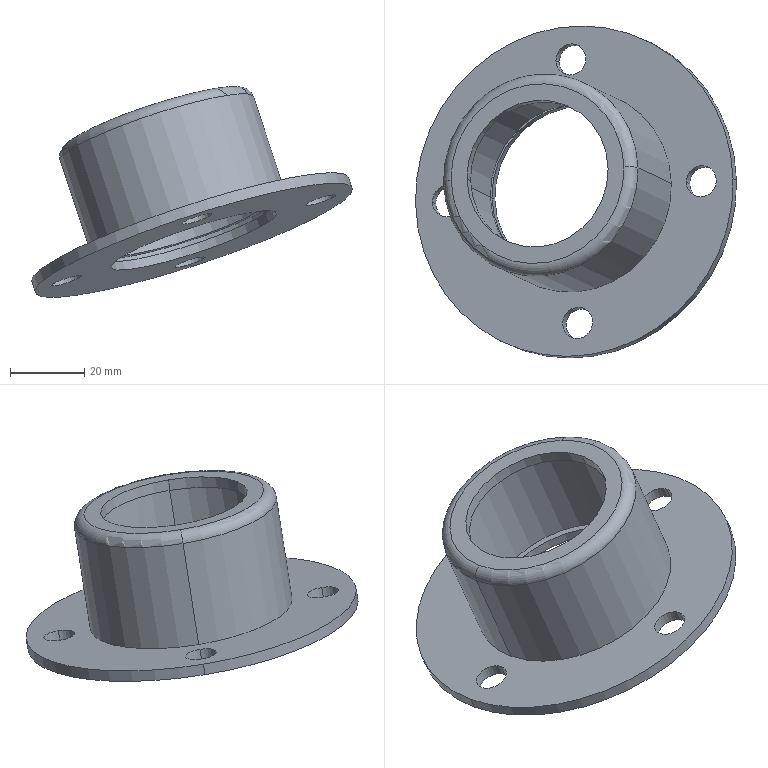Component | SolidWorks | FilmPressingSoilCoveringMechanism2Reverse-2_AttachedSoilDiskAssembly2-1_SoilDiskBearingHousing-1 | 1 solid | 28 faces | box 86.51 x 89.47 x 56.84 mm | volume 34355 mm3 | cylinder 20 | plane 6 | torus 2 | commonest cylinder face diameters 8.5 x8 47 x4 40 x2 55 x2 90 x2 51 x2
STEP:
#1=COLOUR_RGB('',0.7922,0.8196,0.9333);
#2=FILL_AREA_STYLE_COLOUR('',#1);
#3=FILL_AREA_STYLE('',(#2));
#4=SURFACE_STYLE_FILL_AREA(#3);
#5=SURFACE_SIDE_STYLE('',(#4));
#6=SURFACE_STYLE_USAGE(.BOTH.,#5);
#7=PRESENTATION_STYLE_ASSIGNMENT((#6));
#8=CARTESIAN_POINT('',(-74.256,-11.758,103.096));
#9=VERTEX_POINT('',#8);
#10=CARTESIAN_POINT('',(-74.574,-11.783,102.995));
#11=VERTEX_POINT('',#10);
#12=CARTESIAN_POINT('',(-74.415,-11.77,103.045));
#13=DIRECTION('',(-0.3093,0.1459,0.9397));
#14=DIRECTION('',(0.02532,-0.9865,0.1615));
#15=AXIS2_PLACEMENT_3D('',#12,#13,#14);
#16=CIRCLE('',#15,0.1673);
#17=EDGE_CURVE('',#9,#11,#16,.T.);
#18=ORIENTED_EDGE('',*,*,#17,.F.);
#19=CARTESIAN_POINT('',(-74.292,-11.741,103.207));
#20=VERTEX_POINT('',#19);
#21=CARTESIAN_POINT('',(-74.256,-11.758,103.096));
#22=DIRECTION('',(-0.3093,0.1459,0.9397));
#23=VECTOR('',#22,39.37);
#24=LINE('',#21,#23);
#25=EDGE_CURVE('',#9,#20,#24,.T.);
#26=ORIENTED_EDGE('',*,*,#25,.T.);
#27=CARTESIAN_POINT('',(-74.61,-11.765,103.106));
#28=VERTEX_POINT('',#27);
#29=CARTESIAN_POINT('',(-74.451,-11.753,103.156));
#30=DIRECTION('',(-0.3093,0.1459,0.9397));
#31=DIRECTION('',(0.02532,-0.9865,0.1615));
#32=AXIS2_PLACEMENT_3D('',#29,#30,#31);
#33=CIRCLE('',#32,0.1673);
#34=EDGE_CURVE('',#20,#28,#33,.T.);
#35=ORIENTED_EDGE('',*,*,#34,.T.);
#36=CARTESIAN_POINT('',(-74.574,-11.783,102.995));
#37=DIRECTION('',(-0.3093,0.1459,0.9397));
#38=VECTOR('',#37,39.37);
#39=LINE('',#36,#38);
#40=EDGE_CURVE('',#11,#28,#39,.T.);
#41=ORIENTED_EDGE('',*,*,#40,.F.);
#42=EDGE_LOOP('',(#18,#26,#35,#41));
#43=FACE_OUTER_BOUND('',#42,.T.);
#44=CARTESIAN_POINT('',(-74.415,-11.77,103.045));
#45=DIRECTION('',(-0.3093,0.1459,0.9397));
#46=DIRECTION('',(-0.9506,-0.07375,-0.3015));
#47=AXIS2_PLACEMENT_3D('',#44,#45,#46);
#48=CYLINDRICAL_SURFACE('',#47,0.1673);
#49=ADVANCED_FACE('',(#43),#48,.F.);
#50=CARTESIAN_POINT('',(-75.639,-10.464,102.44));
#51=VERTEX_POINT('',#50);
#52=CARTESIAN_POINT('',(-75.957,-10.489,102.339));
#53=VERTEX_POINT('',#52);
#54=CARTESIAN_POINT('',(-75.798,-10.477,102.389));
#55=DIRECTION('',(-0.3093,0.1459,0.9397));
#56=DIRECTION('',(0.9506,0.07375,0.3015));
#57=AXIS2_PLACEMENT_3D('',#54,#55,#56);
#58=CIRCLE('',#57,0.1673);
#59=EDGE_CURVE('',#51,#53,#58,.T.);
#60=ORIENTED_EDGE('',*,*,#59,.F.);
#61=CARTESIAN_POINT('',(-75.675,-10.447,102.551));
#62=VERTEX_POINT('',#61);
#63=CARTESIAN_POINT('',(-75.639,-10.464,102.44));
#64=DIRECTION('',(-0.3093,0.1459,0.9397));
#65=VECTOR('',#64,39.37);
#66=LINE('',#63,#65);
#67=EDGE_CURVE('',#51,#62,#66,.T.);
#68=ORIENTED_EDGE('',*,*,#67,.T.);
#69=CARTESIAN_POINT('',(-75.993,-10.472,102.45));
#70=VERTEX_POINT('',#69);
#71=CARTESIAN_POINT('',(-75.834,-10.459,102.5));
#72=DIRECTION('',(-0.3093,0.1459,0.9397));
#73=DIRECTION('',(0.9506,0.07375,0.3015));
#74=AXIS2_PLACEMENT_3D('',#71,#72,#73);
#75=CIRCLE('',#74,0.1673);
#76=EDGE_CURVE('',#62,#70,#75,.T.);
#77=ORIENTED_EDGE('',*,*,#76,.T.);
#78=CARTESIAN_POINT('',(-75.957,-10.489,102.339));
#79=DIRECTION('',(-0.3093,0.1459,0.9397));
#80=VECTOR('',#79,39.37);
#81=LINE('',#78,#80);
#82=EDGE_CURVE('',#53,#70,#81,.T.);
#83=ORIENTED_EDGE('',*,*,#82,.F.);
#84=EDGE_LOOP('',(#60,#68,#77,#83));
#85=FACE_OUTER_BOUND('',#84,.T.);
#86=CARTESIAN_POINT('',(-75.798,-10.477,102.389));
#87=DIRECTION('',(-0.3093,0.1459,0.9397));
#88=DIRECTION('',(-0.9506,-0.07375,-0.3015));
#89=AXIS2_PLACEMENT_3D('',#86,#87,#88);
#90=CYLINDRICAL_SURFACE('',#89,0.1673);
#91=ADVANCED_FACE('',(#85),#90,.F.);
#92=CARTESIAN_POINT('',(-76.95,-11.967,102.241));
#93=VERTEX_POINT('',#92);
#94=CARTESIAN_POINT('',(-77.268,-11.992,102.14));
#95=VERTEX_POINT('',#94);
#96=CARTESIAN_POINT('',(-77.109,-11.979,102.191));
#97=DIRECTION('',(-0.3093,0.1459,0.9397));
#98=DIRECTION('',(-0.02532,0.9865,-0.1615));
#99=AXIS2_PLACEMENT_3D('',#96,#97,#98);
#100=CIRCLE('',#99,0.1673);
#101=EDGE_CURVE('',#93,#95,#100,.T.);
#102=ORIENTED_EDGE('',*,*,#101,.F.);
#103=CARTESIAN_POINT('',(-76.987,-11.95,102.352));
#104=VERTEX_POINT('',#103);
#105=CARTESIAN_POINT('',(-76.95,-11.967,102.241));
#106=DIRECTION('',(-0.3093,0.1459,0.9397));
#107=VECTOR('',#106,39.37);
#108=LINE('',#105,#107);
#109=EDGE_CURVE('',#93,#104,#108,.T.);
#110=ORIENTED_EDGE('',*,*,#109,.T.);
#111=CARTESIAN_POINT('',(-77.305,-11.975,102.251));
#112=VERTEX_POINT('',#111);
#113=CARTESIAN_POINT('',(-77.146,-11.962,102.302));
#114=DIRECTION('',(-0.3093,0.1459,0.9397));
#115=DIRECTION('',(-0.02532,0.9865,-0.1615));
#116=AXIS2_PLACEMENT_3D('',#113,#114,#115);
#117=CIRCLE('',#116,0.1673);
#118=EDGE_CURVE('',#104,#112,#117,.T.);
#119=ORIENTED_EDGE('',*,*,#118,.T.);
#120=CARTESIAN_POINT('',(-77.268,-11.992,102.14));
#121=DIRECTION('',(-0.3093,0.1459,0.9397));
#122=VECTOR('',#121,39.37);
#123=LINE('',#120,#122);
#124=EDGE_CURVE('',#95,#112,#123,.T.);
#125=ORIENTED_EDGE('',*,*,#124,.F.);
#126=EDGE_LOOP('',(#102,#110,#119,#125));
#127=FACE_OUTER_BOUND('',#126,.T.);
#128=CARTESIAN_POINT('',(-77.109,-11.979,102.191));
#129=DIRECTION('',(-0.3093,0.1459,0.9397));
#130=DIRECTION('',(-0.9506,-0.07375,-0.3015));
#131=AXIS2_PLACEMENT_3D('',#128,#129,#130);
#132=CYLINDRICAL_SURFACE('',#131,0.1673);
#133=ADVANCED_FACE('',(#127),#132,.F.);
#134=CARTESIAN_POINT('',(-75.567,-13.261,102.897));
#135=VERTEX_POINT('',#134);
#136=CARTESIAN_POINT('',(-75.885,-13.285,102.797));
#137=VERTEX_POINT('',#136);
#138=CARTESIAN_POINT('',(-75.726,-13.273,102.847));
#139=DIRECTION('',(-0.3093,0.1459,0.9397));
#140=DIRECTION('',(-0.9506,-0.07375,-0.3015));
#141=AXIS2_PLACEMENT_3D('',#138,#139,#140);
#142=CIRCLE('',#141,0.1673);
#143=EDGE_CURVE('',#135,#137,#142,.T.);
#144=ORIENTED_EDGE('',*,*,#143,.F.);
#145=CARTESIAN_POINT('',(-75.604,-13.244,103.008));
#146=VERTEX_POINT('',#145);
#147=CARTESIAN_POINT('',(-75.567,-13.261,102.897));
#148=DIRECTION('',(-0.3093,0.1459,0.9397));
#149=VECTOR('',#148,39.37);
#150=LINE('',#147,#149);
#151=EDGE_CURVE('',#135,#146,#150,.T.);
#152=ORIENTED_EDGE('',*,*,#151,.T.);
#153=CARTESIAN_POINT('',(-75.922,-13.268,102.908));
#154=VERTEX_POINT('',#153);
#155=CARTESIAN_POINT('',(-75.763,-13.256,102.958));
#156=DIRECTION('',(-0.3093,0.1459,0.9397));
#157=DIRECTION('',(-0.9506,-0.07375,-0.3015));
#158=AXIS2_PLACEMENT_3D('',#155,#156,#157);
#159=CIRCLE('',#158,0.1673);
#160=EDGE_CURVE('',#146,#154,#159,.T.);
#161=ORIENTED_EDGE('',*,*,#160,.T.);
#162=CARTESIAN_POINT('',(-75.885,-13.285,102.797));
#163=DIRECTION('',(-0.3093,0.1459,0.9397));
#164=VECTOR('',#163,39.37);
#165=LINE('',#162,#164);
#166=EDGE_CURVE('',#137,#154,#165,.T.);
#167=ORIENTED_EDGE('',*,*,#166,.F.);
#168=EDGE_LOOP('',(#144,#152,#161,#167));
#169=FACE_OUTER_BOUND('',#168,.T.);
#170=CARTESIAN_POINT('',(-75.726,-13.273,102.847));
#171=DIRECTION('',(-0.3093,0.1459,0.9397));
#172=DIRECTION('',(-0.9506,-0.07375,-0.3015));
#173=AXIS2_PLACEMENT_3D('',#170,#171,#172);
#174=CYLINDRICAL_SURFACE('',#173,0.1673);
#175=ADVANCED_FACE('',(#169),#174,.F.);
#176=CARTESIAN_POINT('',(-76.937,-11.732,103.676));
#177=VERTEX_POINT('',#176);
#178=CARTESIAN_POINT('',(-75.44,-11.616,104.15));
#179=VERTEX_POINT('',#178);
#180=CARTESIAN_POINT('',(-76.188,-11.674,103.913));
#181=DIRECTION('',(0.3093,-0.1459,-0.9397));
#182=DIRECTION('',(0.9506,0.07375,0.3015));
#183=AXIS2_PLACEMENT_3D('',#180,#181,#182);
#184=CIRCLE('',#183,0.7874);
#185=EDGE_CURVE('',#177,#179,#184,.T.);
#186=ORIENTED_EDGE('',*,*,#185,.F.);
#187=CARTESIAN_POINT('',(-76.9,-11.749,103.565));
#188=VERTEX_POINT('',#187);
#189=CARTESIAN_POINT('',(-76.937,-11.732,103.676));
#190=DIRECTION('',(0.3093,-0.1459,-0.9397));
#191=VECTOR('',#190,39.37);
#192=LINE('',#189,#191);
#193=EDGE_CURVE('',#177,#188,#192,.T.);
#194=ORIENTED_EDGE('',*,*,#193,.T.);
#195=CARTESIAN_POINT('',(-75.403,-11.633,104.039));
#196=VERTEX_POINT('',#195);
#197=CARTESIAN_POINT('',(-76.152,-11.691,103.802));
#198=DIRECTION('',(0.3093,-0.1459,-0.9397));
#199=DIRECTION('',(0.9506,0.07375,0.3015));
#200=AXIS2_PLACEMENT_3D('',#197,#198,#199);
#201=CIRCLE('',#200,0.7874);
#202=EDGE_CURVE('',#188,#196,#201,.T.);
#203=ORIENTED_EDGE('',*,*,#202,.T.);
#204=CARTESIAN_POINT('',(-75.44,-11.616,104.15));
#205=DIRECTION('',(0.3093,-0.1459,-0.9397));
#206=VECTOR('',#205,39.37);
#207=LINE('',#204,#206);
#208=EDGE_CURVE('',#179,#196,#207,.T.);
#209=ORIENTED_EDGE('',*,*,#208,.F.);
#210=EDGE_LOOP('',(#186,#194,#203,#209));
#211=FACE_OUTER_BOUND('',#210,.T.);
#212=CARTESIAN_POINT('',(-76.188,-11.674,103.913));
#213=DIRECTION('',(0.3093,-0.1459,-0.9397));
#214=DIRECTION('',(0.9506,0.07375,0.3015));
#215=AXIS2_PLACEMENT_3D('',#212,#213,#214);
#216=CYLINDRICAL_SURFACE('',#215,0.7874);
#217=ADVANCED_FACE('',(#211),#216,.F.);
#218=CARTESIAN_POINT('',(-75.122,-11.611,104.128));
#219=VERTEX_POINT('',#218);
#220=CARTESIAN_POINT('',(-77.181,-11.771,103.476));
#221=VERTEX_POINT('',#220);
#222=CARTESIAN_POINT('',(-76.152,-11.691,103.802));
#223=DIRECTION('',(0.3093,-0.1459,-0.9397));
#224=DIRECTION('',(-0.9506,-0.07375,-0.3015));
#225=AXIS2_PLACEMENT_3D('',#222,#223,#224);
#226=CIRCLE('',#225,1.083);
#227=EDGE_CURVE('',#219,#221,#226,.T.);
#228=ORIENTED_EDGE('',*,*,#227,.F.);
#229=CARTESIAN_POINT('',(-75.271,-11.603,104.204));
#230=VERTEX_POINT('',#229);
#231=CARTESIAN_POINT('',(-75.235,-11.62,104.093));
#232=DIRECTION('',(0.02532,-0.9865,0.1615));
#233=DIRECTION('',(0.,-0.1616,-0.9869));
#234=AXIS2_PLACEMENT_3D('',#231,#232,#233);
#235=CIRCLE('',#234,0.1181);
#236=EDGE_CURVE('',#219,#230,#235,.T.);
#237=ORIENTED_EDGE('',*,*,#236,.T.);
#238=CARTESIAN_POINT('',(-77.105,-11.745,103.622));
#239=VERTEX_POINT('',#238);
#240=CARTESIAN_POINT('',(-76.188,-11.674,103.913));
#241=DIRECTION('',(-0.3093,0.1459,0.9397));
#242=DIRECTION('',(-0.9506,-0.07375,-0.3015));
#243=AXIS2_PLACEMENT_3D('',#240,#241,#242);
#244=CIRCLE('',#243,0.9646);
#245=EDGE_CURVE('',#239,#230,#244,.T.);
#246=ORIENTED_EDGE('',*,*,#245,.F.);
#247=CARTESIAN_POINT('',(-77.069,-11.762,103.511));
#248=DIRECTION('',(-0.02532,0.9865,-0.1615));
#249=DIRECTION('',(0.,0.1616,0.9869));
#250=AXIS2_PLACEMENT_3D('',#247,#248,#249);
#251=CIRCLE('',#250,0.1181);
#252=EDGE_CURVE('',#221,#239,#251,.T.);
#253=ORIENTED_EDGE('',*,*,#252,.F.);
#254=EDGE_LOOP('',(#228,#237,#246,#253));
#255=FACE_OUTER_BOUND('',#254,.T.);
#256=CARTESIAN_POINT('',(-76.152,-11.691,103.802));
#257=DIRECTION('',(-0.3093,0.1459,0.9397));
#258=DIRECTION('',(-0.9506,-0.07375,-0.3015));
#259=AXIS2_PLACEMENT_3D('',#256,#257,#258);
#260=TOROIDAL_SURFACE('',#259,0.9646,0.1181);
#261=ADVANCED_FACE('',(#255),#260,.T.);
#262=ORIENTED_EDGE('',*,*,#227,.T.);
#263=CARTESIAN_POINT('',(-76.828,-11.937,102.403));
#264=VERTEX_POINT('',#263);
#265=CARTESIAN_POINT('',(-77.217,-11.754,103.586));
#266=DIRECTION('',(0.3093,-0.1459,-0.9397));
#267=VECTOR('',#266,39.37);
#268=LINE('',#265,#267);
#269=EDGE_CURVE('',#221,#264,#268,.T.);
#270=ORIENTED_EDGE('',*,*,#269,.T.);
#271=CARTESIAN_POINT('',(-74.769,-11.778,103.055));
#272=VERTEX_POINT('',#271);
#273=CARTESIAN_POINT('',(-75.798,-11.858,102.729));
#274=DIRECTION('',(0.3093,-0.1459,-0.9397));
#275=DIRECTION('',(0.9506,0.07375,0.3015));
#276=AXIS2_PLACEMENT_3D('',#273,#274,#275);
#277=CIRCLE('',#276,1.083);
#278=EDGE_CURVE('',#272,#264,#277,.T.);
#279=ORIENTED_EDGE('',*,*,#278,.F.);
#280=CARTESIAN_POINT('',(-75.159,-11.594,104.239));
#281=DIRECTION('',(0.3093,-0.1459,-0.9397));
#282=VECTOR('',#281,39.37);
#283=LINE('',#280,#282);
#284=EDGE_CURVE('',#219,#272,#283,.T.);
#285=ORIENTED_EDGE('',*,*,#284,.F.);
#286=EDGE_LOOP('',(#262,#270,#279,#285));
#287=FACE_OUTER_BOUND('',#286,.T.);
#288=CARTESIAN_POINT('',(-76.188,-11.674,103.913));
#289=DIRECTION('',(0.3093,-0.1459,-0.9397));
#290=DIRECTION('',(0.9506,0.07375,0.3015));
#291=AXIS2_PLACEMENT_3D('',#288,#289,#290);
#292=CYLINDRICAL_SURFACE('',#291,1.083);
#293=ADVANCED_FACE('',(#287),#292,.T.);
#294=CARTESIAN_POINT('',(-74.114,-11.727,103.263));
#295=VERTEX_POINT('',#294);
#296=CARTESIAN_POINT('',(-77.483,-11.988,102.195));
#297=VERTEX_POINT('',#296);
#298=CARTESIAN_POINT('',(-75.798,-11.858,102.729));
#299=DIRECTION('',(0.3093,-0.1459,-0.9397));
#300=DIRECTION('',(0.9506,0.07375,0.3015));
#301=AXIS2_PLACEMENT_3D('',#298,#299,#300);
#302=CIRCLE('',#301,1.772);
#303=EDGE_CURVE('',#295,#297,#302,.T.);
#304=ORIENTED_EDGE('',*,*,#303,.T.);
#305=CARTESIAN_POINT('',(-77.446,-12.006,102.084));
#306=VERTEX_POINT('',#305);
#307=CARTESIAN_POINT('',(-77.483,-11.988,102.195));
#308=DIRECTION('',(0.3093,-0.1459,-0.9397));
#309=VECTOR('',#308,39.37);
#310=LINE('',#307,#309);
#311=EDGE_CURVE('',#297,#306,#310,.T.);
#312=ORIENTED_EDGE('',*,*,#311,.T.);
#313=CARTESIAN_POINT('',(-74.078,-11.744,103.152));
#314=VERTEX_POINT('',#313);
#315=CARTESIAN_POINT('',(-75.762,-11.875,102.618));
#316=DIRECTION('',(0.3093,-0.1459,-0.9397));
#317=DIRECTION('',(0.9506,0.07375,0.3015));
#318=AXIS2_PLACEMENT_3D('',#315,#316,#317);
#319=CIRCLE('',#318,1.772);
#320=EDGE_CURVE('',#314,#306,#319,.T.);
#321=ORIENTED_EDGE('',*,*,#320,.F.);
#322=CARTESIAN_POINT('',(-74.114,-11.727,103.263));
#323=DIRECTION('',(0.3093,-0.1459,-0.9397));
#324=VECTOR('',#323,39.37);
#325=LINE('',#322,#324);
#326=EDGE_CURVE('',#295,#314,#325,.T.);
#327=ORIENTED_EDGE('',*,*,#326,.F.);
#328=EDGE_LOOP('',(#304,#312,#321,#327));
#329=FACE_OUTER_BOUND('',#328,.T.);
#330=CARTESIAN_POINT('',(-75.798,-11.858,102.729));
#331=DIRECTION('',(0.3093,-0.1459,-0.9397));
#332=DIRECTION('',(0.9506,0.07375,0.3015));
#333=AXIS2_PLACEMENT_3D('',#330,#331,#332);
#334=CYLINDRICAL_SURFACE('',#333,1.772);
#335=ADVANCED_FACE('',(#329),#334,.T.);
#336=CARTESIAN_POINT('',(-77.031,-11.759,103.523));
#337=VERTEX_POINT('',#336);
#338=CARTESIAN_POINT('',(-75.272,-11.623,104.081));
#339=VERTEX_POINT('',#338);
#340=CARTESIAN_POINT('',(-76.152,-11.691,103.802));
#341=DIRECTION('',(0.3093,-0.1459,-0.9397));
#342=DIRECTION('',(0.9506,0.07375,0.3015));
#343=AXIS2_PLACEMENT_3D('',#340,#341,#342);
#344=CIRCLE('',#343,0.9252);
#345=EDGE_CURVE('',#337,#339,#344,.T.);
#346=ORIENTED_EDGE('',*,*,#345,.F.);
#347=CARTESIAN_POINT('',(-76.69,-11.92,102.487));
#348=VERTEX_POINT('',#347);
#349=CARTESIAN_POINT('',(-77.031,-11.759,103.523));
#350=DIRECTION('',(0.3093,-0.1459,-0.9397));
#351=VECTOR('',#350,39.37);
#352=LINE('',#349,#351);
#353=EDGE_CURVE('',#337,#348,#352,.T.);
#354=ORIENTED_EDGE('',*,*,#353,.T.);
#355=CARTESIAN_POINT('',(-74.931,-11.784,103.045));
#356=VERTEX_POINT('',#355);
#357=CARTESIAN_POINT('',(-75.811,-11.852,102.766));
#358=DIRECTION('',(0.3093,-0.1459,-0.9397));
#359=DIRECTION('',(-0.9506,-0.07375,-0.3015));
#360=AXIS2_PLACEMENT_3D('',#357,#358,#359);
#361=CIRCLE('',#360,0.9252);
#362=EDGE_CURVE('',#348,#356,#361,.T.);
#363=ORIENTED_EDGE('',*,*,#362,.T.);
#364=CARTESIAN_POINT('',(-75.272,-11.623,104.081));
#365=DIRECTION('',(0.3093,-0.1459,-0.9397));
#366=VECTOR('',#365,39.37);
#367=LINE('',#364,#366);
#368=EDGE_CURVE('',#339,#356,#367,.T.);
#369=ORIENTED_EDGE('',*,*,#368,.F.);
#370=EDGE_LOOP('',(#346,#354,#363,#369));
#371=FACE_OUTER_BOUND('',#370,.T.);
#372=CARTESIAN_POINT('',(-76.152,-11.691,103.802));
#373=DIRECTION('',(0.3093,-0.1459,-0.9397));
#374=DIRECTION('',(0.9506,0.07375,0.3015));
#375=AXIS2_PLACEMENT_3D('',#372,#373,#374);
#376=CYLINDRICAL_SURFACE('',#375,0.9252);
#377=ADVANCED_FACE('',(#371),#376,.F.);
#378=CARTESIAN_POINT('',(-76.765,-11.926,102.463));
#379=VERTEX_POINT('',#378);
#380=CARTESIAN_POINT('',(-74.856,-11.778,103.069));
#381=VERTEX_POINT('',#380);
#382=CARTESIAN_POINT('',(-75.811,-11.852,102.766));
#383=DIRECTION('',(0.3093,-0.1459,-0.9397));
#384=DIRECTION('',(0.9506,0.07375,0.3015));
#385=AXIS2_PLACEMENT_3D('',#382,#383,#384);
#386=CIRCLE('',#385,1.004);
#387=EDGE_CURVE('',#379,#381,#386,.T.);
#388=ORIENTED_EDGE('',*,*,#387,.F.);
#389=CARTESIAN_POINT('',(-76.747,-11.935,102.408));
#390=VERTEX_POINT('',#389);
#391=CARTESIAN_POINT('',(-76.716,-11.949,102.315));
#392=DIRECTION('',(0.3093,-0.1459,-0.9397));
#393=VECTOR('',#392,39.37);
#394=LINE('',#391,#393);
#395=EDGE_CURVE('',#379,#390,#394,.T.);
#396=ORIENTED_EDGE('',*,*,#395,.T.);
#397=CARTESIAN_POINT('',(-74.838,-11.786,103.013));
#398=VERTEX_POINT('',#397);
#399=CARTESIAN_POINT('',(-75.792,-11.861,102.711));
#400=DIRECTION('',(0.3093,-0.1459,-0.9397));
#401=DIRECTION('',(0.9506,0.07375,0.3015));
#402=AXIS2_PLACEMENT_3D('',#399,#400,#401);
#403=CIRCLE('',#402,1.004);
#404=EDGE_CURVE('',#390,#398,#403,.T.);
#405=ORIENTED_EDGE('',*,*,#404,.T.);
#406=CARTESIAN_POINT('',(-74.808,-11.801,102.921));
#407=DIRECTION('',(0.3093,-0.1459,-0.9397));
#408=VECTOR('',#407,39.37);
#409=LINE('',#406,#408);
#410=EDGE_CURVE('',#381,#398,#409,.T.);
#411=ORIENTED_EDGE('',*,*,#410,.F.);
#412=EDGE_LOOP('',(#388,#396,#405,#411));
#413=FACE_OUTER_BOUND('',#412,.T.);
#414=CARTESIAN_POINT('',(-75.762,-11.875,102.618));
#415=DIRECTION('',(0.3093,-0.1459,-0.9397));
#416=DIRECTION('',(0.9506,0.07375,0.3015));
#417=AXIS2_PLACEMENT_3D('',#414,#415,#416);
#418=CYLINDRICAL_SURFACE('',#417,1.004);
#419=ADVANCED_FACE('',(#413),#418,.F.);
#420=CARTESIAN_POINT('',(-74.913,-11.792,102.989));
#421=VERTEX_POINT('',#420);
#422=CARTESIAN_POINT('',(-76.672,-11.929,102.432));
#423=VERTEX_POINT('',#422);
#424=CARTESIAN_POINT('',(-75.792,-11.861,102.711));
#425=DIRECTION('',(-0.3093,0.1459,0.9397));
#426=DIRECTION('',(0.9506,0.07375,0.3015));
#427=AXIS2_PLACEMENT_3D('',#424,#425,#426);
#428=CIRCLE('',#427,0.9252);
#429=EDGE_CURVE('',#421,#423,#428,.T.);
#430=ORIENTED_EDGE('',*,*,#429,.T.);
#431=CARTESIAN_POINT('',(-76.641,-11.943,102.339));
#432=VERTEX_POINT('',#431);
#433=CARTESIAN_POINT('',(-77.031,-11.759,103.523));
#434=DIRECTION('',(0.3093,-0.1459,-0.9397));
#435=VECTOR('',#434,39.37);
#436=LINE('',#433,#435);
#437=EDGE_CURVE('',#423,#432,#436,.T.);
#438=ORIENTED_EDGE('',*,*,#437,.T.);
#439=CARTESIAN_POINT('',(-74.882,-11.807,102.897));
#440=VERTEX_POINT('',#439);
#441=CARTESIAN_POINT('',(-75.762,-11.875,102.618));
#442=DIRECTION('',(0.3093,-0.1459,-0.9397));
#443=DIRECTION('',(0.9506,0.07375,0.3015));
#444=AXIS2_PLACEMENT_3D('',#441,#442,#443);
#445=CIRCLE('',#444,0.9252);
#446=EDGE_CURVE('',#432,#440,#445,.T.);
#447=ORIENTED_EDGE('',*,*,#446,.T.);
#448=CARTESIAN_POINT('',(-75.272,-11.623,104.081));
#449=DIRECTION('',(0.3093,-0.1459,-0.9397));
#450=VECTOR('',#449,39.37);
#451=LINE('',#448,#450);
#452=EDGE_CURVE('',#421,#440,#451,.T.);
#453=ORIENTED_EDGE('',*,*,#452,.F.);
#454=EDGE_LOOP('',(#430,#438,#447,#453));
#455=FACE_OUTER_BOUND('',#454,.T.);
#456=CARTESIAN_POINT('',(-76.152,-11.691,103.802));
#457=DIRECTION('',(0.3093,-0.1459,-0.9397));
#458=DIRECTION('',(0.9506,0.07375,0.3015));
#459=AXIS2_PLACEMENT_3D('',#456,#457,#458);
#460=CYLINDRICAL_SURFACE('',#459,0.9252);
#461=ADVANCED_FACE('',(#455),#460,.F.);
#462=CARTESIAN_POINT('',(-74.415,-11.77,103.045));
#463=DIRECTION('',(-0.3093,0.1459,0.9397));
#464=DIRECTION('',(0.02532,-0.9865,0.1615));
#465=AXIS2_PLACEMENT_3D('',#462,#463,#464);
#466=CIRCLE('',#465,0.1673);
#467=EDGE_CURVE('',#11,#9,#466,.T.);
#468=ORIENTED_EDGE('',*,*,#467,.T.);
#469=ORIENTED_EDGE('',*,*,#17,.T.);
#470=EDGE_LOOP('',(#468,#469));
#471=FACE_BOUND('',#470,.T.);
#472=CARTESIAN_POINT('',(-75.798,-10.477,102.389));
#473=DIRECTION('',(-0.3093,0.1459,0.9397));
#474=DIRECTION('',(0.9506,0.07375,0.3015));
#475=AXIS2_PLACEMENT_3D('',#472,#473,#474);
#476=CIRCLE('',#475,0.1673);
#477=EDGE_CURVE('',#53,#51,#476,.T.);
#478=ORIENTED_EDGE('',*,*,#477,.T.);
#479=ORIENTED_EDGE('',*,*,#59,.T.);
#480=EDGE_LOOP('',(#478,#479));
#481=FACE_BOUND('',#480,.T.);
#482=CARTESIAN_POINT('',(-77.109,-11.979,102.191));
#483=DIRECTION('',(-0.3093,0.1459,0.9397));
#484=DIRECTION('',(-0.02532,0.9865,-0.1615));
#485=AXIS2_PLACEMENT_3D('',#482,#483,#484);
#486=CIRCLE('',#485,0.1673);
#487=EDGE_CURVE('',#95,#93,#486,.T.);
#488=ORIENTED_EDGE('',*,*,#487,.T.);
#489=ORIENTED_EDGE('',*,*,#101,.T.);
#490=EDGE_LOOP('',(#488,#489));
#491=FACE_BOUND('',#490,.T.);
#492=CARTESIAN_POINT('',(-75.726,-13.273,102.847));
#493=DIRECTION('',(-0.3093,0.1459,0.9397));
#494=DIRECTION('',(-0.9506,-0.07375,-0.3015));
#495=AXIS2_PLACEMENT_3D('',#492,#493,#494);
#496=CIRCLE('',#495,0.1673);
#497=EDGE_CURVE('',#137,#135,#496,.T.);
#498=ORIENTED_EDGE('',*,*,#497,.T.);
#499=ORIENTED_EDGE('',*,*,#143,.T.);
#500=EDGE_LOOP('',(#498,#499));
#501=FACE_BOUND('',#500,.T.);
#502=CARTESIAN_POINT('',(-75.762,-11.875,102.618));
#503=DIRECTION('',(0.3093,-0.1459,-0.9397));
#504=DIRECTION('',(0.9506,0.07375,0.3015));
#505=AXIS2_PLACEMENT_3D('',#502,#503,#504);
#506=CIRCLE('',#505,0.9252);
#507=EDGE_CURVE('',#440,#432,#506,.T.);
#508=ORIENTED_EDGE('',*,*,#507,.F.);
#509=ORIENTED_EDGE('',*,*,#446,.F.);
#510=EDGE_LOOP('',(#508,#509));
#511=FACE_BOUND('',#510,.T.);
#512=ORIENTED_EDGE('',*,*,#320,.T.);
#513=CARTESIAN_POINT('',(-75.762,-11.875,102.618));
#514=DIRECTION('',(0.3093,-0.1459,-0.9397));
#515=DIRECTION('',(0.9506,0.07375,0.3015));
#516=AXIS2_PLACEMENT_3D('',#513,#514,#515);
#517=CIRCLE('',#516,1.772);
#518=EDGE_CURVE('',#306,#314,#517,.T.);
#519=ORIENTED_EDGE('',*,*,#518,.T.);
#520=EDGE_LOOP('',(#512,#519));
#521=FACE_OUTER_BOUND('',#520,.T.);
#522=CARTESIAN_POINT('',(-75.762,-11.875,102.618));
#523=DIRECTION('',(-0.3093,0.1459,0.9397));
#524=DIRECTION('',(-0.9506,-0.07375,-0.3015));
#525=AXIS2_PLACEMENT_3D('',#522,#523,#524);
#526=PLANE('',#525);
#527=ADVANCED_FACE('',(#471,#481,#491,#501,#511,#521),#526,.F.);
#528=ORIENTED_EDGE('',*,*,#437,.F.);
#529=CARTESIAN_POINT('',(-75.792,-11.861,102.711));
#530=DIRECTION('',(-0.3093,0.1459,0.9397));
#531=DIRECTION('',(0.9506,0.07375,0.3015));
#532=AXIS2_PLACEMENT_3D('',#529,#530,#531);
#533=CIRCLE('',#532,0.9252);
#534=EDGE_CURVE('',#423,#421,#533,.T.);
#535=ORIENTED_EDGE('',*,*,#534,.T.);
#536=ORIENTED_EDGE('',*,*,#452,.T.);
#537=ORIENTED_EDGE('',*,*,#507,.T.);
#538=EDGE_LOOP('',(#528,#535,#536,#537));
#539=FACE_OUTER_BOUND('',#538,.T.);
#540=CARTESIAN_POINT('',(-76.152,-11.691,103.802));
#541=DIRECTION('',(0.3093,-0.1459,-0.9397));
#542=DIRECTION('',(0.9506,0.07375,0.3015));
#543=AXIS2_PLACEMENT_3D('',#540,#541,#542);
#544=CYLINDRICAL_SURFACE('',#543,0.9252);
#545=ADVANCED_FACE('',(#539),#544,.F.);
#546=CARTESIAN_POINT('',(-75.811,-11.852,102.766));
#547=DIRECTION('',(0.3093,-0.1459,-0.9397));
#548=DIRECTION('',(0.9506,0.07375,0.3015));
#549=AXIS2_PLACEMENT_3D('',#546,#547,#548);
#550=CIRCLE('',#549,1.004);
#551=EDGE_CURVE('',#381,#379,#550,.T.);
#552=ORIENTED_EDGE('',*,*,#551,.T.);
#553=ORIENTED_EDGE('',*,*,#387,.T.);
#554=EDGE_LOOP('',(#552,#553));
#555=FACE_OUTER_BOUND('',#554,.T.);
#556=CARTESIAN_POINT('',(-75.811,-11.852,102.766));
#557=DIRECTION('',(0.3093,-0.1459,-0.9397));
#558=DIRECTION('',(-0.9506,-0.07375,-0.3015));
#559=AXIS2_PLACEMENT_3D('',#556,#557,#558);
#560=CIRCLE('',#559,0.9252);
#561=EDGE_CURVE('',#356,#348,#560,.T.);
#562=ORIENTED_EDGE('',*,*,#561,.F.);
#563=ORIENTED_EDGE('',*,*,#362,.F.);
#564=EDGE_LOOP('',(#562,#563));
#565=FACE_BOUND('',#564,.T.);
#566=CARTESIAN_POINT('',(-74.856,-11.778,103.069));
#567=DIRECTION('',(-0.3093,0.1459,0.9397));
#568=DIRECTION('',(-0.9506,-0.07375,-0.3015));
#569=AXIS2_PLACEMENT_3D('',#566,#567,#568);
#570=PLANE('',#569);
#571=ADVANCED_FACE('',(#555,#565),#570,.F.);
#572=CARTESIAN_POINT('',(-75.792,-11.861,102.711));
#573=DIRECTION('',(0.3093,-0.1459,-0.9397));
#574=DIRECTION('',(0.9506,0.07375,0.3015));
#575=AXIS2_PLACEMENT_3D('',#572,#573,#574);
#576=CIRCLE('',#575,1.004);
#577=EDGE_CURVE('',#398,#390,#576,.T.);
#578=ORIENTED_EDGE('',*,*,#577,.F.);
#579=ORIENTED_EDGE('',*,*,#404,.F.);
#580=EDGE_LOOP('',(#578,#579));
#581=FACE_OUTER_BOUND('',#580,.T.);
#582=ORIENTED_EDGE('',*,*,#429,.F.);
#583=ORIENTED_EDGE('',*,*,#534,.F.);
#584=EDGE_LOOP('',(#582,#583));
#585=FACE_BOUND('',#584,.T.);
#586=CARTESIAN_POINT('',(-74.838,-11.786,103.013));
#587=DIRECTION('',(0.3093,-0.1459,-0.9397));
#588=DIRECTION('',(0.9506,0.07375,0.3015));
#589=AXIS2_PLACEMENT_3D('',#586,#587,#588);
#590=PLANE('',#589);
#591=ADVANCED_FACE('',(#581,#585),#590,.F.);
#592=ORIENTED_EDGE('',*,*,#395,.F.);
#593=ORIENTED_EDGE('',*,*,#551,.F.);
#594=ORIENTED_EDGE('',*,*,#410,.T.);
#595=ORIENTED_EDGE('',*,*,#577,.T.);
#596=EDGE_LOOP('',(#592,#593,#594,#595));
#597=FACE_OUTER_BOUND('',#596,.T.);
#598=CARTESIAN_POINT('',(-75.762,-11.875,102.618));
#599=DIRECTION('',(0.3093,-0.1459,-0.9397));
#600=DIRECTION('',(0.9506,0.07375,0.3015));
#601=AXIS2_PLACEMENT_3D('',#598,#599,#600);
#602=CYLINDRICAL_SURFACE('',#601,1.004);
#603=ADVANCED_FACE('',(#597),#602,.F.);
#604=CARTESIAN_POINT('',(-76.152,-11.691,103.802));
#605=DIRECTION('',(0.3093,-0.1459,-0.9397));
#606=DIRECTION('',(0.9506,0.07375,0.3015));
#607=AXIS2_PLACEMENT_3D('',#604,#605,#606);
#608=CIRCLE('',#607,0.7874);
#609=EDGE_CURVE('',#196,#188,#608,.T.);
#610=ORIENTED_EDGE('',*,*,#609,.F.);
#611=ORIENTED_EDGE('',*,*,#202,.F.);
#612=EDGE_LOOP('',(#610,#611));
#613=FACE_BOUND('',#612,.T.);
#614=CARTESIAN_POINT('',(-76.152,-11.691,103.802));
#615=DIRECTION('',(0.3093,-0.1459,-0.9397));
#616=DIRECTION('',(0.9506,0.07375,0.3015));
#617=AXIS2_PLACEMENT_3D('',#614,#615,#616);
#618=CIRCLE('',#617,0.9252);
#619=EDGE_CURVE('',#339,#337,#618,.T.);
#620=ORIENTED_EDGE('',*,*,#619,.T.);
#621=ORIENTED_EDGE('',*,*,#345,.T.);
#622=EDGE_LOOP('',(#620,#621));
#623=FACE_OUTER_BOUND('',#622,.T.);
#624=CARTESIAN_POINT('',(-76.152,-11.691,103.802));
#625=DIRECTION('',(0.3093,-0.1459,-0.9397));
#626=DIRECTION('',(0.9506,0.07375,0.3015));
#627=AXIS2_PLACEMENT_3D('',#624,#625,#626);
#628=PLANE('',#627);
#629=ADVANCED_FACE('',(#613,#623),#628,.T.);
#630=ORIENTED_EDGE('',*,*,#353,.F.);
#631=ORIENTED_EDGE('',*,*,#619,.F.);
#632=ORIENTED_EDGE('',*,*,#368,.T.);
#633=ORIENTED_EDGE('',*,*,#561,.T.);
#634=EDGE_LOOP('',(#630,#631,#632,#633));
#635=FACE_OUTER_BOUND('',#634,.T.);
#636=CARTESIAN_POINT('',(-76.152,-11.691,103.802));
#637=DIRECTION('',(0.3093,-0.1459,-0.9397));
#638=DIRECTION('',(0.9506,0.07375,0.3015));
#639=AXIS2_PLACEMENT_3D('',#636,#637,#638);
#640=CYLINDRICAL_SURFACE('',#639,0.9252);
#641=ADVANCED_FACE('',(#635),#640,.F.);
#642=ORIENTED_EDGE('',*,*,#311,.F.);
#643=CARTESIAN_POINT('',(-75.798,-11.858,102.729));
#644=DIRECTION('',(0.3093,-0.1459,-0.9397));
#645=DIRECTION('',(0.9506,0.07375,0.3015));
#646=AXIS2_PLACEMENT_3D('',#643,#644,#645);
#647=CIRCLE('',#646,1.772);
#648=EDGE_CURVE('',#297,#295,#647,.T.);
#649=ORIENTED_EDGE('',*,*,#648,.T.);
#650=ORIENTED_EDGE('',*,*,#326,.T.);
#651=ORIENTED_EDGE('',*,*,#518,.F.);
#652=EDGE_LOOP('',(#642,#649,#650,#651));
#653=FACE_OUTER_BOUND('',#652,.T.);
#654=CARTESIAN_POINT('',(-75.798,-11.858,102.729));
#655=DIRECTION('',(0.3093,-0.1459,-0.9397));
#656=DIRECTION('',(0.9506,0.07375,0.3015));
#657=AXIS2_PLACEMENT_3D('',#654,#655,#656);
#658=CYLINDRICAL_SURFACE('',#657,1.772);
#659=ADVANCED_FACE('',(#653),#658,.T.);
#660=CARTESIAN_POINT('',(-74.451,-11.753,103.156));
#661=DIRECTION('',(-0.3093,0.1459,0.9397));
#662=DIRECTION('',(0.02532,-0.9865,0.1615));
#663=AXIS2_PLACEMENT_3D('',#660,#661,#662);
#664=CIRCLE('',#663,0.1673);
#665=EDGE_CURVE('',#28,#20,#664,.T.);
#666=ORIENTED_EDGE('',*,*,#665,.F.);
#667=ORIENTED_EDGE('',*,*,#34,.F.);
#668=EDGE_LOOP('',(#666,#667));
#669=FACE_BOUND('',#668,.T.);
#670=CARTESIAN_POINT('',(-75.834,-10.459,102.5));
#671=DIRECTION('',(-0.3093,0.1459,0.9397));
#672=DIRECTION('',(0.9506,0.07375,0.3015));
#673=AXIS2_PLACEMENT_3D('',#670,#671,#672);
#674=CIRCLE('',#673,0.1673);
#675=EDGE_CURVE('',#70,#62,#674,.T.);
#676=ORIENTED_EDGE('',*,*,#675,.F.);
#677=ORIENTED_EDGE('',*,*,#76,.F.);
#678=EDGE_LOOP('',(#676,#677));
#679=FACE_BOUND('',#678,.T.);
#680=CARTESIAN_POINT('',(-77.146,-11.962,102.302));
#681=DIRECTION('',(-0.3093,0.1459,0.9397));
#682=DIRECTION('',(-0.02532,0.9865,-0.1615));
#683=AXIS2_PLACEMENT_3D('',#680,#681,#682);
#684=CIRCLE('',#683,0.1673);
#685=EDGE_CURVE('',#112,#104,#684,.T.);
#686=ORIENTED_EDGE('',*,*,#685,.F.);
#687=ORIENTED_EDGE('',*,*,#118,.F.);
#688=EDGE_LOOP('',(#686,#687));
#689=FACE_BOUND('',#688,.T.);
#690=CARTESIAN_POINT('',(-75.763,-13.256,102.958));
#691=DIRECTION('',(-0.3093,0.1459,0.9397));
#692=DIRECTION('',(-0.9506,-0.07375,-0.3015));
#693=AXIS2_PLACEMENT_3D('',#690,#691,#692);
#694=CIRCLE('',#693,0.1673);
#695=EDGE_CURVE('',#154,#146,#694,.T.);
#696=ORIENTED_EDGE('',*,*,#695,.F.);
#697=ORIENTED_EDGE('',*,*,#160,.F.);
#698=EDGE_LOOP('',(#696,#697));
#699=FACE_BOUND('',#698,.T.);
#700=ORIENTED_EDGE('',*,*,#278,.T.);
#701=CARTESIAN_POINT('',(-75.798,-11.858,102.729));
#702=DIRECTION('',(0.3093,-0.1459,-0.9397));
#703=DIRECTION('',(0.9506,0.07375,0.3015));
#704=AXIS2_PLACEMENT_3D('',#701,#702,#703);
#705=CIRCLE('',#704,1.083);
#706=EDGE_CURVE('',#264,#272,#705,.T.);
#707=ORIENTED_EDGE('',*,*,#706,.T.);
#708=EDGE_LOOP('',(#700,#707));
#709=FACE_BOUND('',#708,.T.);
#710=ORIENTED_EDGE('',*,*,#303,.F.);
#711=ORIENTED_EDGE('',*,*,#648,.F.);
#712=EDGE_LOOP('',(#710,#711));
#713=FACE_OUTER_BOUND('',#712,.T.);
#714=CARTESIAN_POINT('',(-75.798,-11.858,102.729));
#715=DIRECTION('',(0.3093,-0.1459,-0.9397));
#716=DIRECTION('',(0.9506,0.07375,0.3015));
#717=AXIS2_PLACEMENT_3D('',#714,#715,#716);
#718=PLANE('',#717);
#719=ADVANCED_FACE('',(#669,#679,#689,#699,#709,#713),#718,.F.);
#720=CARTESIAN_POINT('',(-76.188,-11.674,103.913));
#721=DIRECTION('',(0.3093,-0.1459,-0.9397));
#722=DIRECTION('',(0.9506,0.07375,0.3015));
#723=AXIS2_PLACEMENT_3D('',#720,#721,#722);
#724=CIRCLE('',#723,0.7874);
#725=EDGE_CURVE('',#179,#177,#724,.T.);
#726=ORIENTED_EDGE('',*,*,#725,.T.);
#727=ORIENTED_EDGE('',*,*,#185,.T.);
#728=EDGE_LOOP('',(#726,#727));
#729=FACE_BOUND('',#728,.T.);
#730=ORIENTED_EDGE('',*,*,#245,.T.);
#731=CARTESIAN_POINT('',(-76.188,-11.674,103.913));
#732=DIRECTION('',(-0.3093,0.1459,0.9397));
#733=DIRECTION('',(-0.9506,-0.07375,-0.3015));
#734=AXIS2_PLACEMENT_3D('',#731,#732,#733);
#735=CIRCLE('',#734,0.9646);
#736=EDGE_CURVE('',#230,#239,#735,.T.);
#737=ORIENTED_EDGE('',*,*,#736,.T.);
#738=EDGE_LOOP('',(#730,#737));
#739=FACE_OUTER_BOUND('',#738,.T.);
#740=CARTESIAN_POINT('',(-76.188,-11.674,103.913));
#741=DIRECTION('',(-0.3093,0.1459,0.9397));
#742=DIRECTION('',(-0.9506,-0.07375,-0.3015));
#743=AXIS2_PLACEMENT_3D('',#740,#741,#742);
#744=PLANE('',#743);
#745=ADVANCED_FACE('',(#729,#739),#744,.T.);
#746=ORIENTED_EDGE('',*,*,#269,.F.);
#747=CARTESIAN_POINT('',(-76.152,-11.691,103.802));
#748=DIRECTION('',(0.3093,-0.1459,-0.9397));
#749=DIRECTION('',(-0.9506,-0.07375,-0.3015));
#750=AXIS2_PLACEMENT_3D('',#747,#748,#749);
#751=CIRCLE('',#750,1.083);
#752=EDGE_CURVE('',#221,#219,#751,.T.);
#753=ORIENTED_EDGE('',*,*,#752,.T.);
#754=ORIENTED_EDGE('',*,*,#284,.T.);
#755=ORIENTED_EDGE('',*,*,#706,.F.);
#756=EDGE_LOOP('',(#746,#753,#754,#755));
#757=FACE_OUTER_BOUND('',#756,.T.);
#758=CARTESIAN_POINT('',(-76.188,-11.674,103.913));
#759=DIRECTION('',(0.3093,-0.1459,-0.9397));
#760=DIRECTION('',(0.9506,0.07375,0.3015));
#761=AXIS2_PLACEMENT_3D('',#758,#759,#760);
#762=CYLINDRICAL_SURFACE('',#761,1.083);
#763=ADVANCED_FACE('',(#757),#762,.T.);
#764=ORIENTED_EDGE('',*,*,#236,.F.);
#765=ORIENTED_EDGE('',*,*,#752,.F.);
#766=ORIENTED_EDGE('',*,*,#252,.T.);
#767=ORIENTED_EDGE('',*,*,#736,.F.);
#768=EDGE_LOOP('',(#764,#765,#766,#767));
#769=FACE_OUTER_BOUND('',#768,.T.);
#770=CARTESIAN_POINT('',(-76.152,-11.691,103.802));
#771=DIRECTION('',(-0.3093,0.1459,0.9397));
#772=DIRECTION('',(-0.9506,-0.07375,-0.3015));
#773=AXIS2_PLACEMENT_3D('',#770,#771,#772);
#774=TOROIDAL_SURFACE('',#773,0.9646,0.1181);
#775=ADVANCED_FACE('',(#769),#774,.T.);
#776=ORIENTED_EDGE('',*,*,#193,.F.);
#777=ORIENTED_EDGE('',*,*,#725,.F.);
#778=ORIENTED_EDGE('',*,*,#208,.T.);
#779=ORIENTED_EDGE('',*,*,#609,.T.);
#780=EDGE_LOOP('',(#776,#777,#778,#779));
#781=FACE_OUTER_BOUND('',#780,.T.);
#782=CARTESIAN_POINT('',(-76.188,-11.674,103.913));
#783=DIRECTION('',(0.3093,-0.1459,-0.9397));
#784=DIRECTION('',(0.9506,0.07375,0.3015));
#785=AXIS2_PLACEMENT_3D('',#782,#783,#784);
#786=CYLINDRICAL_SURFACE('',#785,0.7874);
#787=ADVANCED_FACE('',(#781),#786,.F.);
#788=ORIENTED_EDGE('',*,*,#151,.F.);
#789=ORIENTED_EDGE('',*,*,#497,.F.);
#790=ORIENTED_EDGE('',*,*,#166,.T.);
#791=ORIENTED_EDGE('',*,*,#695,.T.);
#792=EDGE_LOOP('',(#788,#789,#790,#791));
#793=FACE_OUTER_BOUND('',#792,.T.);
#794=CARTESIAN_POINT('',(-75.726,-13.273,102.847));
#795=DIRECTION('',(-0.3093,0.1459,0.9397));
#796=DIRECTION('',(-0.9506,-0.07375,-0.3015));
#797=AXIS2_PLACEMENT_3D('',#794,#795,#796);
#798=CYLINDRICAL_SURFACE('',#797,0.1673);
#799=ADVANCED_FACE('',(#793),#798,.F.);
#800=ORIENTED_EDGE('',*,*,#109,.F.);
#801=ORIENTED_EDGE('',*,*,#487,.F.);
#802=ORIENTED_EDGE('',*,*,#124,.T.);
#803=ORIENTED_EDGE('',*,*,#685,.T.);
#804=EDGE_LOOP('',(#800,#801,#802,#803));
#805=FACE_OUTER_BOUND('',#804,.T.);
#806=CARTESIAN_POINT('',(-77.109,-11.979,102.191));
#807=DIRECTION('',(-0.3093,0.1459,0.9397));
#808=DIRECTION('',(-0.9506,-0.07375,-0.3015));
#809=AXIS2_PLACEMENT_3D('',#806,#807,#808);
#810=CYLINDRICAL_SURFACE('',#809,0.1673);
#811=ADVANCED_FACE('',(#805),#810,.F.);
#812=ORIENTED_EDGE('',*,*,#67,.F.);
#813=ORIENTED_EDGE('',*,*,#477,.F.);
#814=ORIENTED_EDGE('',*,*,#82,.T.);
#815=ORIENTED_EDGE('',*,*,#675,.T.);
#816=EDGE_LOOP('',(#812,#813,#814,#815));
#817=FACE_OUTER_BOUND('',#816,.T.);
#818=CARTESIAN_POINT('',(-75.798,-10.477,102.389));
#819=DIRECTION('',(-0.3093,0.1459,0.9397));
#820=DIRECTION('',(-0.9506,-0.07375,-0.3015));
#821=AXIS2_PLACEMENT_3D('',#818,#819,#820);
#822=CYLINDRICAL_SURFACE('',#821,0.1673);
#823=ADVANCED_FACE('',(#817),#822,.F.);
#824=ORIENTED_EDGE('',*,*,#25,.F.);
#825=ORIENTED_EDGE('',*,*,#467,.F.);
#826=ORIENTED_EDGE('',*,*,#40,.T.);
#827=ORIENTED_EDGE('',*,*,#665,.T.);
#828=EDGE_LOOP('',(#824,#825,#826,#827));
#829=FACE_OUTER_BOUND('',#828,.T.);
#830=CARTESIAN_POINT('',(-74.415,-11.77,103.045));
#831=DIRECTION('',(-0.3093,0.1459,0.9397));
#832=DIRECTION('',(-0.9506,-0.07375,-0.3015));
#833=AXIS2_PLACEMENT_3D('',#830,#831,#832);
#834=CYLINDRICAL_SURFACE('',#833,0.1673);
#835=ADVANCED_FACE('',(#829),#834,.F.);
#836=CLOSED_SHELL('',(#49,#91,#133,#175,#217,#261,#293,#335,#377,#419,#461,#527,#545,#571,#591,#603,#629,#641,#659,#719,#745,#763,#775,#787,#799,#811,#823,#835));
#837=MANIFOLD_SOLID_BREP('',#836);
#838=STYLED_ITEM('',(#7),#837);
#839=(LENGTH_UNIT()NAMED_UNIT(*)SI_UNIT($,.METRE.));
#840=LENGTH_MEASURE_WITH_UNIT(LENGTH_MEASURE(0.0254),#839);
#841=DIMENSIONAL_EXPONENTS(1.,0.,0.,0.,0.,0.,0.);
#842=(CONVERSION_BASED_UNIT('',#840)LENGTH_UNIT()NAMED_UNIT(#841));
#843=UNCERTAINTY_MEASURE_WITH_UNIT(LENGTH_MEASURE(0.00001),#842,'','');
#844=(NAMED_UNIT(*)PLANE_ANGLE_UNIT()SI_UNIT($,.RADIAN.));
#845=(NAMED_UNIT(*)SI_UNIT($,.STERADIAN.)SOLID_ANGLE_UNIT());
#846=(GEOMETRIC_REPRESENTATION_CONTEXT(3)GLOBAL_UNCERTAINTY_ASSIGNED_CONTEXT((#843))GLOBAL_UNIT_ASSIGNED_CONTEXT((#842,#844,#845))REPRESENTATION_CONTEXT('',''));
#847=MECHANICAL_DESIGN_GEOMETRIC_PRESENTATION_REPRESENTATION('',(#838),#846);
#848=PRESENTATION_LAYER_ASSIGNMENT('','',(#838));
#849=CARTESIAN_POINT('',(0.,0.,0.));
#850=DIRECTION('',(0.,0.,1.));
#851=DIRECTION('',(1.,0.,0.));
#852=AXIS2_PLACEMENT_3D('',#849,#850,#851);
#853=(LENGTH_UNIT()NAMED_UNIT(*)SI_UNIT($,.METRE.));
#854=LENGTH_MEASURE_WITH_UNIT(LENGTH_MEASURE(0.0254),#853);
#855=DIMENSIONAL_EXPONENTS(1.,0.,0.,0.,0.,0.,0.);
#856=(CONVERSION_BASED_UNIT('',#854)LENGTH_UNIT()NAMED_UNIT(#855));
#857=UNCERTAINTY_MEASURE_WITH_UNIT(LENGTH_MEASURE(0.00001),#856,'','');
#858=(NAMED_UNIT(*)PLANE_ANGLE_UNIT()SI_UNIT($,.RADIAN.));
#859=(NAMED_UNIT(*)SI_UNIT($,.STERADIAN.)SOLID_ANGLE_UNIT());
#860=(GEOMETRIC_REPRESENTATION_CONTEXT(3)GLOBAL_UNCERTAINTY_ASSIGNED_CONTEXT((#857))GLOBAL_UNIT_ASSIGNED_CONTEXT((#856,#858,#859))REPRESENTATION_CONTEXT('',''));
#861=ADVANCED_BREP_SHAPE_REPRESENTATION('',(#837,#852),#860);